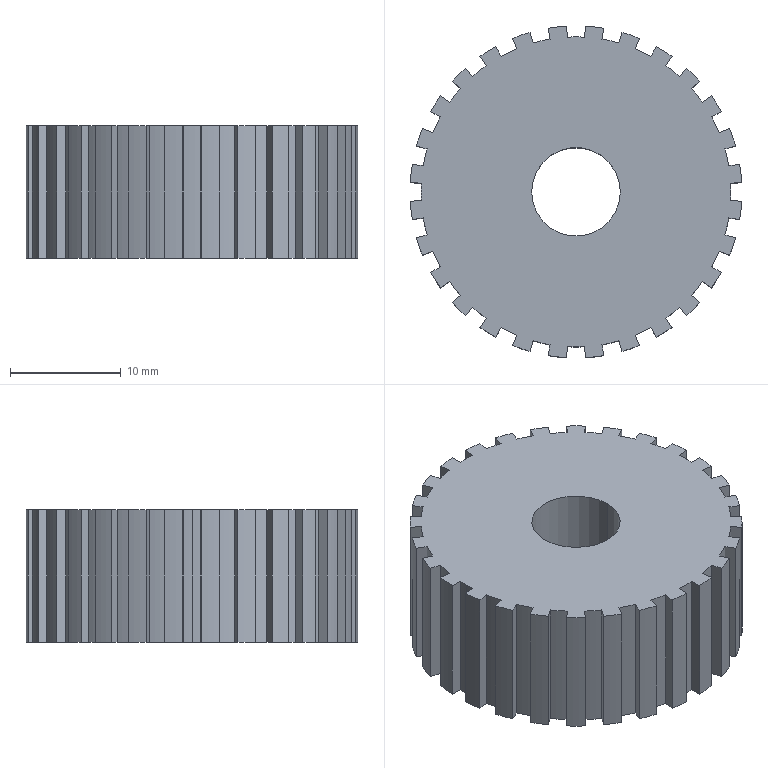Component | SolidWorks | Pulley11.1-2 | 1 solid | 117 faces | box 29.95 x 29.95 x 12 mm | volume 7332 mm3 | cylinder 59 | plane 58 | commonest cylinder face diameters 28 x29 30 x28 8 x2
build123d program:
from build123d import *

# Parameters (mm, degrees)
SKETCH1_2_R         = 4
BOSS_EXTRUDE1_DEPTH = 6


with BuildPart() as part:
    # Sketch1_2 → Boss-Extrude1 (new, symmetric)
    with BuildSketch(Plane.XY):
        with BuildLine():
            Line((13.978, -0.785), (14.976, -0.8411))
            ThreePointArc((14.976, -0.8411), (14.906, -1.679), (14.788, -2.513))
            Line((14.788, -2.513), (13.802, -2.345))
            ThreePointArc((13.802, -2.345), (13.649, -3.115), (13.453, -3.876))
            Line((13.453, -3.876), (14.414, -4.153))
            ThreePointArc((14.414, -4.153), (14.158, -4.954), (13.858, -5.74))
            Line((13.858, -5.74), (12.934, -5.358))
            ThreePointArc((12.934, -5.358), (12.614, -6.074), (12.253, -6.772))
            Line((12.253, -6.772), (13.128, -7.256))
            ThreePointArc((13.128, -7.256), (12.701, -7.98), (12.233, -8.68))
            Line((12.233, -8.68), (11.418, -8.101))
            ThreePointArc((11.418, -8.101), (10.946, -8.729), (10.439, -9.329))
            Line((10.439, -9.329), (11.185, -9.995))
            ThreePointArc((11.185, -9.995), (10.607, -10.607), (9.995, -11.185))
            Line((9.995, -11.185), (9.329, -10.439))
            ThreePointArc((9.329, -10.439), (8.729, -10.946), (8.101, -11.418))
            Line((8.101, -11.418), (8.68, -12.233))
            ThreePointArc((8.68, -12.233), (7.98, -12.701), (7.256, -13.128))
            Line((7.256, -13.128), (6.772, -12.253))
            ThreePointArc((6.772, -12.253), (6.074, -12.614), (5.358, -12.934))
            Line((5.358, -12.934), (5.74, -13.858))
            ThreePointArc((5.74, -13.858), (4.954, -14.158), (4.153, -14.414))
            Line((4.153, -14.414), (3.876, -13.453))
            ThreePointArc((3.876, -13.453), (3.115, -13.649), (2.345, -13.802))
            Line((2.345, -13.802), (2.513, -14.788))
            ThreePointArc((2.513, -14.788), (1.679, -14.906), (0.8411, -14.976))
            Line((0.8411, -14.976), (0.785, -13.978))
            ThreePointArc((0.785, -13.978), (0, -14), (-0.785, -13.978))
            Line((-0.785, -13.978), (-0.8411, -14.976))
            ThreePointArc((-0.8411, -14.976), (-1.679, -14.906), (-2.513, -14.788))
            Line((-2.513, -14.788), (-2.345, -13.802))
            ThreePointArc((-2.345, -13.802), (-3.115, -13.649), (-3.876, -13.453))
            Line((-3.876, -13.453), (-4.153, -14.414))
            ThreePointArc((-4.153, -14.414), (-4.954, -14.158), (-5.74, -13.858))
            Line((-5.74, -13.858), (-5.358, -12.934))
            ThreePointArc((-5.358, -12.934), (-6.074, -12.614), (-6.772, -12.253))
            Line((-6.772, -12.253), (-7.256, -13.128))
            ThreePointArc((-7.256, -13.128), (-7.98, -12.701), (-8.68, -12.233))
            Line((-8.68, -12.233), (-8.101, -11.418))
            ThreePointArc((-8.101, -11.418), (-8.729, -10.946), (-9.329, -10.439))
            Line((-9.329, -10.439), (-9.995, -11.185))
            ThreePointArc((-9.995, -11.185), (-10.607, -10.607), (-11.185, -9.995))
            Line((-11.185, -9.995), (-10.439, -9.329))
            ThreePointArc((-10.439, -9.329), (-10.946, -8.729), (-11.418, -8.101))
            Line((-11.418, -8.101), (-12.233, -8.68))
            ThreePointArc((-12.233, -8.68), (-12.701, -7.98), (-13.128, -7.256))
            Line((-13.128, -7.256), (-12.253, -6.772))
            ThreePointArc((-12.253, -6.772), (-12.614, -6.074), (-12.934, -5.358))
            Line((-12.934, -5.358), (-13.858, -5.74))
            ThreePointArc((-13.858, -5.74), (-14.158, -4.954), (-14.414, -4.153))
            Line((-14.414, -4.153), (-13.453, -3.876))
            ThreePointArc((-13.453, -3.876), (-13.649, -3.115), (-13.802, -2.345))
            Line((-13.802, -2.345), (-14.788, -2.513))
            ThreePointArc((-14.788, -2.513), (-14.906, -1.679), (-14.976, -0.8411))
            Line((-14.976, -0.8411), (-13.978, -0.785))
            ThreePointArc((-13.978, -0.785), (-14, 0), (-13.978, 0.785))
            Line((-13.978, 0.785), (-14.976, 0.8411))
            ThreePointArc((-14.976, 0.8411), (-14.906, 1.679), (-14.788, 2.513))
            Line((-14.788, 2.513), (-13.802, 2.345))
            ThreePointArc((-13.802, 2.345), (-13.649, 3.115), (-13.453, 3.876))
            Line((-13.453, 3.876), (-14.414, 4.153))
            ThreePointArc((-14.414, 4.153), (-14.158, 4.954), (-13.858, 5.74))
            Line((-13.858, 5.74), (-12.934, 5.358))
            ThreePointArc((-12.934, 5.358), (-12.614, 6.074), (-12.253, 6.772))
            Line((-12.253, 6.772), (-13.128, 7.256))
            ThreePointArc((-13.128, 7.256), (-12.701, 7.98), (-12.233, 8.68))
            Line((-12.233, 8.68), (-11.418, 8.101))
            ThreePointArc((-11.418, 8.101), (-10.946, 8.729), (-10.439, 9.329))
            Line((-10.439, 9.329), (-11.185, 9.995))
            ThreePointArc((-11.185, 9.995), (-10.607, 10.607), (-9.995, 11.185))
            Line((-9.995, 11.185), (-9.329, 10.439))
            ThreePointArc((-9.329, 10.439), (-8.729, 10.946), (-8.101, 11.418))
            Line((-8.101, 11.418), (-8.68, 12.233))
            ThreePointArc((-8.68, 12.233), (-7.98, 12.701), (-7.256, 13.128))
            Line((-7.256, 13.128), (-6.772, 12.253))
            ThreePointArc((-6.772, 12.253), (-6.074, 12.614), (-5.358, 12.934))
            Line((-5.358, 12.934), (-5.74, 13.858))
            ThreePointArc((-5.74, 13.858), (-4.954, 14.158), (-4.153, 14.414))
            Line((-4.153, 14.414), (-3.876, 13.453))
            ThreePointArc((-3.876, 13.453), (-3.115, 13.649), (-2.345, 13.802))
            Line((-2.345, 13.802), (-2.513, 14.788))
            ThreePointArc((-2.513, 14.788), (-1.679, 14.906), (-0.8411, 14.976))
            Line((-0.8411, 14.976), (-0.785, 13.978))
            ThreePointArc((-0.785, 13.978), (0, 14), (0.785, 13.978))
            Line((0.785, 13.978), (0.8411, 14.976))
            ThreePointArc((0.8411, 14.976), (1.679, 14.906), (2.513, 14.788))
            Line((2.513, 14.788), (2.345, 13.802))
            ThreePointArc((2.345, 13.802), (3.115, 13.649), (3.876, 13.453))
            Line((3.876, 13.453), (4.153, 14.414))
            ThreePointArc((4.153, 14.414), (4.954, 14.158), (5.74, 13.858))
            Line((5.74, 13.858), (5.358, 12.934))
            ThreePointArc((5.358, 12.934), (6.074, 12.614), (6.772, 12.253))
            Line((6.772, 12.253), (7.256, 13.128))
            ThreePointArc((7.256, 13.128), (7.98, 12.701), (8.68, 12.233))
            Line((8.68, 12.233), (8.101, 11.418))
            ThreePointArc((8.101, 11.418), (8.729, 10.946), (9.329, 10.439))
            Line((9.329, 10.439), (9.995, 11.185))
            ThreePointArc((9.995, 11.185), (10.607, 10.607), (11.185, 9.995))
            Line((11.185, 9.995), (10.439, 9.329))
            ThreePointArc((10.439, 9.329), (10.946, 8.729), (11.418, 8.101))
            Line((11.418, 8.101), (12.233, 8.68))
            ThreePointArc((12.233, 8.68), (12.701, 7.98), (13.128, 7.256))
            Line((13.128, 7.256), (12.253, 6.772))
            ThreePointArc((12.253, 6.772), (12.614, 6.074), (12.934, 5.358))
            Line((12.934, 5.358), (13.858, 5.74))
            ThreePointArc((13.858, 5.74), (14.158, 4.954), (14.414, 4.153))
            Line((14.414, 4.153), (13.453, 3.876))
            ThreePointArc((13.453, 3.876), (13.649, 3.115), (13.802, 2.345))
            Line((13.802, 2.345), (14.788, 2.513))
            ThreePointArc((14.788, 2.513), (14.906, 1.679), (14.976, 0.8411))
            Line((14.976, 0.8411), (13.978, 0.785))
            ThreePointArc((13.978, 0.785), (14, 0), (13.978, -0.785))
        make_face()
        Circle(SKETCH1_2_R, mode=Mode.SUBTRACT)
    extrude(amount=BOSS_EXTRUDE1_DEPTH, both=True)


solid = part.part

# Placed as in the assembly
solid = solid.moved(Location((40.5, 135, -94), (0, 0, 0)))